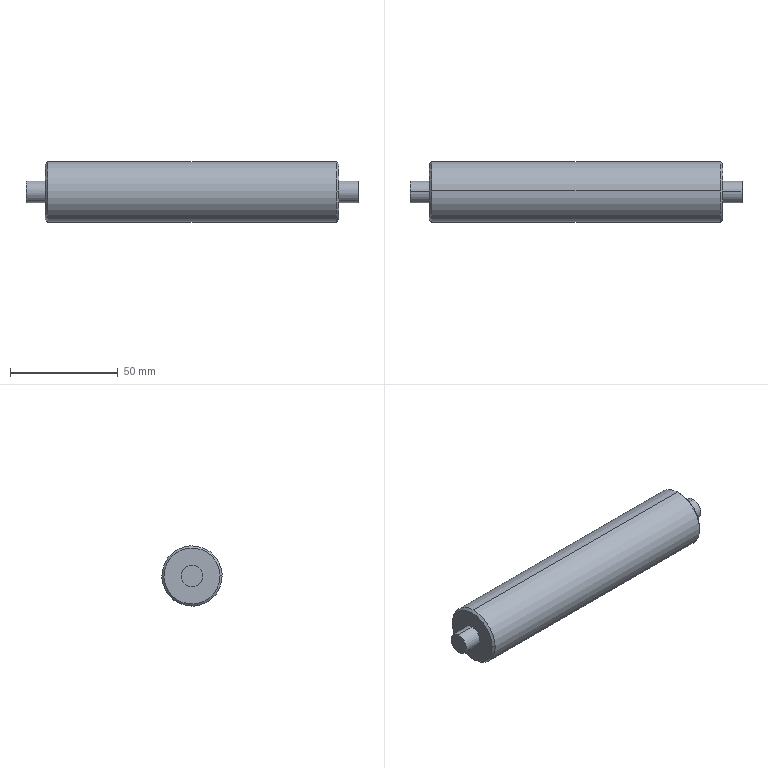Component | SolidWorks | Roller-1 | 1 solid | 14 faces | box 154 x 28 x 28 mm | volume 85070 mm3 | cylinder 6 | cone 4 | plane 4 | commonest cylinder face diameters 10 x4 28 x2
build123d program:
from build123d import *

# Parameters (mm, degrees)
CHAMFER1_SIZE = 1


with BuildPart() as part:
    # Sketch1 → Revolve1 (revolve)
    with BuildSketch(Plane.XY):
        Polygon((3, 77), (8, 77), (8, 68), (17, 68), (17, -68), (8, -68), (8, -77), (3, -77), align=None)
    revolve(axis=Axis((3, -77, 0), (0, 1, 0)))

    # Chamfer1
    chamfer1_edges = [part.edges().sort_by_distance(p)[0] for p in [
        (-11, -68, 0),
        (-11, 68, 0),
    ]]
    chamfer(chamfer1_edges, length=CHAMFER1_SIZE)


solid = part.part

# Placed as in the assembly
solid = solid.moved(Location((192.398, 352.813, 160), (0, 0, 90)))
STEP:
#1=COLOUR_RGB('',0.7922,0.8196,0.9333);
#2=FILL_AREA_STYLE_COLOUR('',#1);
#3=FILL_AREA_STYLE('',(#2));
#4=SURFACE_STYLE_FILL_AREA(#3);
#5=SURFACE_SIDE_STYLE('',(#4));
#6=SURFACE_STYLE_USAGE(.BOTH.,#5);
#7=PRESENTATION_STYLE_ASSIGNMENT((#6));
#8=CARTESIAN_POINT('',(4.898,13.497,6.316));
#9=VERTEX_POINT('',#8);
#10=CARTESIAN_POINT('',(4.898,14.52,6.282));
#11=VERTEX_POINT('',#10);
#12=CARTESIAN_POINT('',(4.898,14.008,6.299));
#13=DIRECTION('',(-1.,0.,-0.));
#14=DIRECTION('',(0.,-0.03369,-0.9994));
#15=AXIS2_PLACEMENT_3D('',#12,#13,#14);
#16=CIRCLE('',#15,0.5118);
#17=EDGE_CURVE('',#9,#11,#16,.T.);
#18=ORIENTED_EDGE('',*,*,#17,.F.);
#19=CARTESIAN_POINT('',(4.937,13.458,6.318));
#20=VERTEX_POINT('',#19);
#21=CARTESIAN_POINT('',(4.937,13.458,6.318));
#22=DIRECTION('',(0.7071,-0.7067,0.02382));
#23=VECTOR('',#22,39.37);
#24=LINE('',#21,#23);
#25=EDGE_CURVE('',#9,#20,#24,.T.);
#26=ORIENTED_EDGE('',*,*,#25,.T.);
#27=CARTESIAN_POINT('',(4.937,14.027,6.85));
#28=VERTEX_POINT('',#27);
#29=CARTESIAN_POINT('',(4.937,14.008,6.299));
#30=DIRECTION('',(1.,-0.,0.));
#31=DIRECTION('',(0.,-0.9994,0.03369));
#32=AXIS2_PLACEMENT_3D('',#29,#30,#31);
#33=CIRCLE('',#32,0.5512);
#34=EDGE_CURVE('',#28,#20,#33,.T.);
#35=ORIENTED_EDGE('',*,*,#34,.F.);
#36=CARTESIAN_POINT('',(4.937,14.559,6.281));
#37=VERTEX_POINT('',#36);
#38=CARTESIAN_POINT('',(4.937,14.008,6.299));
#39=DIRECTION('',(1.,-0.,0.));
#40=DIRECTION('',(0.,-0.9994,0.03369));
#41=AXIS2_PLACEMENT_3D('',#38,#39,#40);
#42=CIRCLE('',#41,0.5512);
#43=EDGE_CURVE('',#37,#28,#42,.T.);
#44=ORIENTED_EDGE('',*,*,#43,.F.);
#45=CARTESIAN_POINT('',(4.937,14.559,6.281));
#46=DIRECTION('',(0.7071,0.7067,-0.02382));
#47=VECTOR('',#46,39.37);
#48=LINE('',#45,#47);
#49=EDGE_CURVE('',#11,#37,#48,.T.);
#50=ORIENTED_EDGE('',*,*,#49,.F.);
#51=EDGE_LOOP('',(#18,#26,#35,#44,#50));
#52=FACE_OUTER_BOUND('',#51,.T.);
#53=CARTESIAN_POINT('',(4.937,14.008,6.299));
#54=DIRECTION('',(1.,-0.,0.));
#55=DIRECTION('',(0.,0.9994,-0.03369));
#56=AXIS2_PLACEMENT_3D('',#53,#54,#55);
#57=CONICAL_SURFACE('',#56,0.5512,0.7854);
#58=ADVANCED_FACE('',(#52),#57,.T.);
#59=CARTESIAN_POINT('',(10.252,14.52,6.282));
#60=VERTEX_POINT('',#59);
#61=CARTESIAN_POINT('',(10.252,13.497,6.316));
#62=VERTEX_POINT('',#61);
#63=CARTESIAN_POINT('',(10.252,14.008,6.299));
#64=DIRECTION('',(1.,-0.,0.));
#65=DIRECTION('',(0.,0.03369,0.9994));
#66=AXIS2_PLACEMENT_3D('',#63,#64,#65);
#67=CIRCLE('',#66,0.5118);
#68=EDGE_CURVE('',#60,#62,#67,.T.);
#69=ORIENTED_EDGE('',*,*,#68,.F.);
#70=CARTESIAN_POINT('',(10.213,14.559,6.281));
#71=VERTEX_POINT('',#70);
#72=CARTESIAN_POINT('',(10.252,14.52,6.282));
#73=DIRECTION('',(-0.7071,0.7067,-0.02382));
#74=VECTOR('',#73,39.37);
#75=LINE('',#72,#74);
#76=EDGE_CURVE('',#60,#71,#75,.T.);
#77=ORIENTED_EDGE('',*,*,#76,.T.);
#78=CARTESIAN_POINT('',(10.213,14.027,6.85));
#79=VERTEX_POINT('',#78);
#80=CARTESIAN_POINT('',(10.213,14.008,6.299));
#81=DIRECTION('',(-1.,0.,-0.));
#82=DIRECTION('',(0.,0.9994,-0.03369));
#83=AXIS2_PLACEMENT_3D('',#80,#81,#82);
#84=CIRCLE('',#83,0.5512);
#85=EDGE_CURVE('',#79,#71,#84,.T.);
#86=ORIENTED_EDGE('',*,*,#85,.F.);
#87=CARTESIAN_POINT('',(10.213,13.458,6.318));
#88=VERTEX_POINT('',#87);
#89=CARTESIAN_POINT('',(10.213,14.008,6.299));
#90=DIRECTION('',(-1.,0.,-0.));
#91=DIRECTION('',(0.,0.9994,-0.03369));
#92=AXIS2_PLACEMENT_3D('',#89,#90,#91);
#93=CIRCLE('',#92,0.5512);
#94=EDGE_CURVE('',#88,#79,#93,.T.);
#95=ORIENTED_EDGE('',*,*,#94,.F.);
#96=CARTESIAN_POINT('',(10.252,13.497,6.316));
#97=DIRECTION('',(-0.7071,-0.7067,0.02382));
#98=VECTOR('',#97,39.37);
#99=LINE('',#96,#98);
#100=EDGE_CURVE('',#62,#88,#99,.T.);
#101=ORIENTED_EDGE('',*,*,#100,.F.);
#102=EDGE_LOOP('',(#69,#77,#86,#95,#101));
#103=FACE_OUTER_BOUND('',#102,.T.);
#104=CARTESIAN_POINT('',(10.252,14.008,6.299));
#105=DIRECTION('',(-1.,0.,-0.));
#106=DIRECTION('',(0.,-0.9994,0.03369));
#107=AXIS2_PLACEMENT_3D('',#104,#105,#106);
#108=CONICAL_SURFACE('',#107,0.5118,0.7854);
#109=ADVANCED_FACE('',(#103),#108,.T.);
#110=CARTESIAN_POINT('',(10.252,14.015,6.496));
#111=VERTEX_POINT('',#110);
#112=CARTESIAN_POINT('',(10.252,14.002,6.102));
#113=VERTEX_POINT('',#112);
#114=CARTESIAN_POINT('',(10.252,14.008,6.299));
#115=DIRECTION('',(1.,-0.,0.));
#116=DIRECTION('',(0.,0.03369,0.9994));
#117=AXIS2_PLACEMENT_3D('',#114,#115,#116);
#118=CIRCLE('',#117,0.1969);
#119=EDGE_CURVE('',#111,#113,#118,.T.);
#120=ORIENTED_EDGE('',*,*,#119,.T.);
#121=CARTESIAN_POINT('',(10.606,14.002,6.102));
#122=VERTEX_POINT('',#121);
#123=CARTESIAN_POINT('',(10.606,14.002,6.102));
#124=DIRECTION('',(1.,-0.,0.));
#125=VECTOR('',#124,39.37);
#126=LINE('',#123,#125);
#127=EDGE_CURVE('',#113,#122,#126,.T.);
#128=ORIENTED_EDGE('',*,*,#127,.T.);
#129=CARTESIAN_POINT('',(10.606,14.015,6.496));
#130=VERTEX_POINT('',#129);
#131=CARTESIAN_POINT('',(10.606,14.008,6.299));
#132=DIRECTION('',(1.,-0.,0.));
#133=DIRECTION('',(0.,0.03369,0.9994));
#134=AXIS2_PLACEMENT_3D('',#131,#132,#133);
#135=CIRCLE('',#134,0.1969);
#136=EDGE_CURVE('',#130,#122,#135,.T.);
#137=ORIENTED_EDGE('',*,*,#136,.F.);
#138=CARTESIAN_POINT('',(10.606,14.015,6.496));
#139=DIRECTION('',(1.,-0.,0.));
#140=VECTOR('',#139,39.37);
#141=LINE('',#138,#140);
#142=EDGE_CURVE('',#111,#130,#141,.T.);
#143=ORIENTED_EDGE('',*,*,#142,.F.);
#144=EDGE_LOOP('',(#120,#128,#137,#143));
#145=FACE_OUTER_BOUND('',#144,.T.);
#146=CARTESIAN_POINT('',(10.606,14.008,6.299));
#147=DIRECTION('',(1.,-0.,0.));
#148=DIRECTION('',(0.,0.03369,0.9994));
#149=AXIS2_PLACEMENT_3D('',#146,#147,#148);
#150=CYLINDRICAL_SURFACE('',#149,0.1969);
#151=ADVANCED_FACE('',(#145),#150,.T.);
#152=ORIENTED_EDGE('',*,*,#34,.T.);
#153=CARTESIAN_POINT('',(4.937,13.99,5.748));
#154=VERTEX_POINT('',#153);
#155=CARTESIAN_POINT('',(4.937,14.008,6.299));
#156=DIRECTION('',(1.,-0.,0.));
#157=DIRECTION('',(0.,-0.9994,0.03369));
#158=AXIS2_PLACEMENT_3D('',#155,#156,#157);
#159=CIRCLE('',#158,0.5512);
#160=EDGE_CURVE('',#20,#154,#159,.T.);
#161=ORIENTED_EDGE('',*,*,#160,.T.);
#162=CARTESIAN_POINT('',(10.213,13.99,5.748));
#163=VERTEX_POINT('',#162);
#164=CARTESIAN_POINT('',(10.606,13.99,5.748));
#165=DIRECTION('',(1.,-0.,0.));
#166=VECTOR('',#165,39.37);
#167=LINE('',#164,#166);
#168=EDGE_CURVE('',#154,#163,#167,.T.);
#169=ORIENTED_EDGE('',*,*,#168,.T.);
#170=CARTESIAN_POINT('',(10.213,14.008,6.299));
#171=DIRECTION('',(-1.,0.,-0.));
#172=DIRECTION('',(0.,0.9994,-0.03369));
#173=AXIS2_PLACEMENT_3D('',#170,#171,#172);
#174=CIRCLE('',#173,0.5512);
#175=EDGE_CURVE('',#163,#88,#174,.T.);
#176=ORIENTED_EDGE('',*,*,#175,.T.);
#177=ORIENTED_EDGE('',*,*,#94,.T.);
#178=CARTESIAN_POINT('',(10.606,14.027,6.85));
#179=DIRECTION('',(1.,-0.,0.));
#180=VECTOR('',#179,39.37);
#181=LINE('',#178,#180);
#182=EDGE_CURVE('',#28,#79,#181,.T.);
#183=ORIENTED_EDGE('',*,*,#182,.F.);
#184=EDGE_LOOP('',(#152,#161,#169,#176,#177,#183));
#185=FACE_OUTER_BOUND('',#184,.T.);
#186=CARTESIAN_POINT('',(10.606,14.008,6.299));
#187=DIRECTION('',(1.,-0.,0.));
#188=DIRECTION('',(0.,0.03369,0.9994));
#189=AXIS2_PLACEMENT_3D('',#186,#187,#188);
#190=CYLINDRICAL_SURFACE('',#189,0.5512);
#191=ADVANCED_FACE('',(#185),#190,.T.);
#192=CARTESIAN_POINT('',(4.543,14.015,6.496));
#193=VERTEX_POINT('',#192);
#194=CARTESIAN_POINT('',(4.543,14.002,6.102));
#195=VERTEX_POINT('',#194);
#196=CARTESIAN_POINT('',(4.543,14.008,6.299));
#197=DIRECTION('',(1.,-0.,0.));
#198=DIRECTION('',(0.,0.03369,0.9994));
#199=AXIS2_PLACEMENT_3D('',#196,#197,#198);
#200=CIRCLE('',#199,0.1969);
#201=EDGE_CURVE('',#193,#195,#200,.T.);
#202=ORIENTED_EDGE('',*,*,#201,.T.);
#203=CARTESIAN_POINT('',(4.898,14.002,6.102));
#204=VERTEX_POINT('',#203);
#205=CARTESIAN_POINT('',(10.606,14.002,6.102));
#206=DIRECTION('',(1.,-0.,0.));
#207=VECTOR('',#206,39.37);
#208=LINE('',#205,#207);
#209=EDGE_CURVE('',#195,#204,#208,.T.);
#210=ORIENTED_EDGE('',*,*,#209,.T.);
#211=CARTESIAN_POINT('',(4.898,14.015,6.496));
#212=VERTEX_POINT('',#211);
#213=CARTESIAN_POINT('',(4.898,14.008,6.299));
#214=DIRECTION('',(1.,-0.,0.));
#215=DIRECTION('',(0.,0.03369,0.9994));
#216=AXIS2_PLACEMENT_3D('',#213,#214,#215);
#217=CIRCLE('',#216,0.1969);
#218=EDGE_CURVE('',#212,#204,#217,.T.);
#219=ORIENTED_EDGE('',*,*,#218,.F.);
#220=CARTESIAN_POINT('',(10.606,14.015,6.496));
#221=DIRECTION('',(1.,-0.,0.));
#222=VECTOR('',#221,39.37);
#223=LINE('',#220,#222);
#224=EDGE_CURVE('',#193,#212,#223,.T.);
#225=ORIENTED_EDGE('',*,*,#224,.F.);
#226=EDGE_LOOP('',(#202,#210,#219,#225));
#227=FACE_OUTER_BOUND('',#226,.T.);
#228=CARTESIAN_POINT('',(10.606,14.008,6.299));
#229=DIRECTION('',(1.,-0.,0.));
#230=DIRECTION('',(0.,0.03369,0.9994));
#231=AXIS2_PLACEMENT_3D('',#228,#229,#230);
#232=CYLINDRICAL_SURFACE('',#231,0.1969);
#233=ADVANCED_FACE('',(#227),#232,.T.);
#234=ORIENTED_EDGE('',*,*,#201,.F.);
#235=CARTESIAN_POINT('',(4.543,14.008,6.299));
#236=DIRECTION('',(1.,-0.,0.));
#237=DIRECTION('',(0.,0.03369,0.9994));
#238=AXIS2_PLACEMENT_3D('',#235,#236,#237);
#239=CIRCLE('',#238,0.1969);
#240=EDGE_CURVE('',#195,#193,#239,.T.);
#241=ORIENTED_EDGE('',*,*,#240,.F.);
#242=EDGE_LOOP('',(#234,#241));
#243=FACE_OUTER_BOUND('',#242,.T.);
#244=CARTESIAN_POINT('',(4.543,14.008,6.299));
#245=DIRECTION('',(-1.,0.,-0.));
#246=DIRECTION('',(0.,-0.03369,-0.9994));
#247=AXIS2_PLACEMENT_3D('',#244,#245,#246);
#248=PLANE('',#247);
#249=ADVANCED_FACE('',(#243),#248,.T.);
#250=ORIENTED_EDGE('',*,*,#209,.F.);
#251=ORIENTED_EDGE('',*,*,#240,.T.);
#252=ORIENTED_EDGE('',*,*,#224,.T.);
#253=CARTESIAN_POINT('',(4.898,14.008,6.299));
#254=DIRECTION('',(1.,-0.,0.));
#255=DIRECTION('',(0.,0.03369,0.9994));
#256=AXIS2_PLACEMENT_3D('',#253,#254,#255);
#257=CIRCLE('',#256,0.1969);
#258=EDGE_CURVE('',#204,#212,#257,.T.);
#259=ORIENTED_EDGE('',*,*,#258,.F.);
#260=EDGE_LOOP('',(#250,#251,#252,#259));
#261=FACE_OUTER_BOUND('',#260,.T.);
#262=CARTESIAN_POINT('',(10.606,14.008,6.299));
#263=DIRECTION('',(1.,-0.,0.));
#264=DIRECTION('',(0.,0.03369,0.9994));
#265=AXIS2_PLACEMENT_3D('',#262,#263,#264);
#266=CYLINDRICAL_SURFACE('',#265,0.1969);
#267=ADVANCED_FACE('',(#261),#266,.T.);
#268=CARTESIAN_POINT('',(4.898,14.008,6.299));
#269=DIRECTION('',(-1.,0.,-0.));
#270=DIRECTION('',(0.,-0.03369,-0.9994));
#271=AXIS2_PLACEMENT_3D('',#268,#269,#270);
#272=CIRCLE('',#271,0.5118);
#273=EDGE_CURVE('',#11,#9,#272,.T.);
#274=ORIENTED_EDGE('',*,*,#273,.T.);
#275=ORIENTED_EDGE('',*,*,#17,.T.);
#276=EDGE_LOOP('',(#274,#275));
#277=FACE_OUTER_BOUND('',#276,.T.);
#278=ORIENTED_EDGE('',*,*,#218,.T.);
#279=ORIENTED_EDGE('',*,*,#258,.T.);
#280=EDGE_LOOP('',(#278,#279));
#281=FACE_BOUND('',#280,.T.);
#282=CARTESIAN_POINT('',(4.898,14.015,6.496));
#283=DIRECTION('',(-1.,0.,-0.));
#284=DIRECTION('',(0.,-0.03369,-0.9994));
#285=AXIS2_PLACEMENT_3D('',#282,#283,#284);
#286=PLANE('',#285);
#287=ADVANCED_FACE('',(#277,#281),#286,.T.);
#288=ORIENTED_EDGE('',*,*,#168,.F.);
#289=CARTESIAN_POINT('',(4.937,14.008,6.299));
#290=DIRECTION('',(1.,-0.,0.));
#291=DIRECTION('',(0.,-0.9994,0.03369));
#292=AXIS2_PLACEMENT_3D('',#289,#290,#291);
#293=CIRCLE('',#292,0.5512);
#294=EDGE_CURVE('',#154,#37,#293,.T.);
#295=ORIENTED_EDGE('',*,*,#294,.T.);
#296=ORIENTED_EDGE('',*,*,#43,.T.);
#297=ORIENTED_EDGE('',*,*,#182,.T.);
#298=ORIENTED_EDGE('',*,*,#85,.T.);
#299=CARTESIAN_POINT('',(10.213,14.008,6.299));
#300=DIRECTION('',(-1.,0.,-0.));
#301=DIRECTION('',(0.,0.9994,-0.03369));
#302=AXIS2_PLACEMENT_3D('',#299,#300,#301);
#303=CIRCLE('',#302,0.5512);
#304=EDGE_CURVE('',#71,#163,#303,.T.);
#305=ORIENTED_EDGE('',*,*,#304,.T.);
#306=EDGE_LOOP('',(#288,#295,#296,#297,#298,#305));
#307=FACE_OUTER_BOUND('',#306,.T.);
#308=CARTESIAN_POINT('',(10.606,14.008,6.299));
#309=DIRECTION('',(1.,-0.,0.));
#310=DIRECTION('',(0.,0.03369,0.9994));
#311=AXIS2_PLACEMENT_3D('',#308,#309,#310);
#312=CYLINDRICAL_SURFACE('',#311,0.5512);
#313=ADVANCED_FACE('',(#307),#312,.T.);
#314=CARTESIAN_POINT('',(10.252,14.008,6.299));
#315=DIRECTION('',(1.,-0.,0.));
#316=DIRECTION('',(0.,0.03369,0.9994));
#317=AXIS2_PLACEMENT_3D('',#314,#315,#316);
#318=CIRCLE('',#317,0.5118);
#319=EDGE_CURVE('',#62,#60,#318,.T.);
#320=ORIENTED_EDGE('',*,*,#319,.T.);
#321=ORIENTED_EDGE('',*,*,#68,.T.);
#322=EDGE_LOOP('',(#320,#321));
#323=FACE_OUTER_BOUND('',#322,.T.);
#324=ORIENTED_EDGE('',*,*,#119,.F.);
#325=CARTESIAN_POINT('',(10.252,14.008,6.299));
#326=DIRECTION('',(1.,-0.,0.));
#327=DIRECTION('',(0.,0.03369,0.9994));
#328=AXIS2_PLACEMENT_3D('',#325,#326,#327);
#329=CIRCLE('',#328,0.1969);
#330=EDGE_CURVE('',#113,#111,#329,.T.);
#331=ORIENTED_EDGE('',*,*,#330,.F.);
#332=EDGE_LOOP('',(#324,#331));
#333=FACE_BOUND('',#332,.T.);
#334=CARTESIAN_POINT('',(10.252,14.027,6.85));
#335=DIRECTION('',(1.,-0.,0.));
#336=DIRECTION('',(-0.,0.03369,0.9994));
#337=AXIS2_PLACEMENT_3D('',#334,#335,#336);
#338=PLANE('',#337);
#339=ADVANCED_FACE('',(#323,#333),#338,.T.);
#340=ORIENTED_EDGE('',*,*,#127,.F.);
#341=ORIENTED_EDGE('',*,*,#330,.T.);
#342=ORIENTED_EDGE('',*,*,#142,.T.);
#343=CARTESIAN_POINT('',(10.606,14.008,6.299));
#344=DIRECTION('',(1.,-0.,0.));
#345=DIRECTION('',(0.,0.03369,0.9994));
#346=AXIS2_PLACEMENT_3D('',#343,#344,#345);
#347=CIRCLE('',#346,0.1969);
#348=EDGE_CURVE('',#122,#130,#347,.T.);
#349=ORIENTED_EDGE('',*,*,#348,.F.);
#350=EDGE_LOOP('',(#340,#341,#342,#349));
#351=FACE_OUTER_BOUND('',#350,.T.);
#352=CARTESIAN_POINT('',(10.606,14.008,6.299));
#353=DIRECTION('',(1.,-0.,0.));
#354=DIRECTION('',(0.,0.03369,0.9994));
#355=AXIS2_PLACEMENT_3D('',#352,#353,#354);
#356=CYLINDRICAL_SURFACE('',#355,0.1969);
#357=ADVANCED_FACE('',(#351),#356,.T.);
#358=ORIENTED_EDGE('',*,*,#136,.T.);
#359=ORIENTED_EDGE('',*,*,#348,.T.);
#360=EDGE_LOOP('',(#358,#359));
#361=FACE_OUTER_BOUND('',#360,.T.);
#362=CARTESIAN_POINT('',(10.606,14.015,6.496));
#363=DIRECTION('',(1.,-0.,0.));
#364=DIRECTION('',(-0.,0.03369,0.9994));
#365=AXIS2_PLACEMENT_3D('',#362,#363,#364);
#366=PLANE('',#365);
#367=ADVANCED_FACE('',(#361),#366,.T.);
#368=ORIENTED_EDGE('',*,*,#76,.F.);
#369=ORIENTED_EDGE('',*,*,#319,.F.);
#370=ORIENTED_EDGE('',*,*,#100,.T.);
#371=ORIENTED_EDGE('',*,*,#175,.F.);
#372=ORIENTED_EDGE('',*,*,#304,.F.);
#373=EDGE_LOOP('',(#368,#369,#370,#371,#372));
#374=FACE_OUTER_BOUND('',#373,.T.);
#375=CARTESIAN_POINT('',(10.252,14.008,6.299));
#376=DIRECTION('',(-1.,0.,-0.));
#377=DIRECTION('',(0.,-0.9994,0.03369));
#378=AXIS2_PLACEMENT_3D('',#375,#376,#377);
#379=CONICAL_SURFACE('',#378,0.5118,0.7854);
#380=ADVANCED_FACE('',(#374),#379,.T.);
#381=ORIENTED_EDGE('',*,*,#25,.F.);
#382=ORIENTED_EDGE('',*,*,#273,.F.);
#383=ORIENTED_EDGE('',*,*,#49,.T.);
#384=ORIENTED_EDGE('',*,*,#294,.F.);
#385=ORIENTED_EDGE('',*,*,#160,.F.);
#386=EDGE_LOOP('',(#381,#382,#383,#384,#385));
#387=FACE_OUTER_BOUND('',#386,.T.);
#388=CARTESIAN_POINT('',(4.937,14.008,6.299));
#389=DIRECTION('',(1.,-0.,0.));
#390=DIRECTION('',(0.,0.9994,-0.03369));
#391=AXIS2_PLACEMENT_3D('',#388,#389,#390);
#392=CONICAL_SURFACE('',#391,0.5512,0.7854);
#393=ADVANCED_FACE('',(#387),#392,.T.);
#394=CLOSED_SHELL('',(#58,#109,#151,#191,#233,#249,#267,#287,#313,#339,#357,#367,#380,#393));
#395=MANIFOLD_SOLID_BREP('',#394);
#396=STYLED_ITEM('',(#7),#395);
#397=(LENGTH_UNIT()NAMED_UNIT(*)SI_UNIT($,.METRE.));
#398=LENGTH_MEASURE_WITH_UNIT(LENGTH_MEASURE(0.0254),#397);
#399=DIMENSIONAL_EXPONENTS(1.,0.,0.,0.,0.,0.,0.);
#400=(CONVERSION_BASED_UNIT('',#398)LENGTH_UNIT()NAMED_UNIT(#399));
#401=UNCERTAINTY_MEASURE_WITH_UNIT(LENGTH_MEASURE(0.00001),#400,'','');
#402=(NAMED_UNIT(*)PLANE_ANGLE_UNIT()SI_UNIT($,.RADIAN.));
#403=(NAMED_UNIT(*)SI_UNIT($,.STERADIAN.)SOLID_ANGLE_UNIT());
#404=(GEOMETRIC_REPRESENTATION_CONTEXT(3)GLOBAL_UNCERTAINTY_ASSIGNED_CONTEXT((#401))GLOBAL_UNIT_ASSIGNED_CONTEXT((#400,#402,#403))REPRESENTATION_CONTEXT('',''));
#405=MECHANICAL_DESIGN_GEOMETRIC_PRESENTATION_REPRESENTATION('',(#396),#404);
#406=PRESENTATION_LAYER_ASSIGNMENT('','',(#396));
#407=CARTESIAN_POINT('',(0.,0.,0.));
#408=DIRECTION('',(0.,0.,1.));
#409=DIRECTION('',(1.,0.,0.));
#410=AXIS2_PLACEMENT_3D('',#407,#408,#409);
#411=(LENGTH_UNIT()NAMED_UNIT(*)SI_UNIT($,.METRE.));
#412=LENGTH_MEASURE_WITH_UNIT(LENGTH_MEASURE(0.0254),#411);
#413=DIMENSIONAL_EXPONENTS(1.,0.,0.,0.,0.,0.,0.);
#414=(CONVERSION_BASED_UNIT('',#412)LENGTH_UNIT()NAMED_UNIT(#413));
#415=UNCERTAINTY_MEASURE_WITH_UNIT(LENGTH_MEASURE(0.00001),#414,'','');
#416=(NAMED_UNIT(*)PLANE_ANGLE_UNIT()SI_UNIT($,.RADIAN.));
#417=(NAMED_UNIT(*)SI_UNIT($,.STERADIAN.)SOLID_ANGLE_UNIT());
#418=(GEOMETRIC_REPRESENTATION_CONTEXT(3)GLOBAL_UNCERTAINTY_ASSIGNED_CONTEXT((#415))GLOBAL_UNIT_ASSIGNED_CONTEXT((#414,#416,#417))REPRESENTATION_CONTEXT('',''));
#419=ADVANCED_BREP_SHAPE_REPRESENTATION('',(#395,#410),#418);